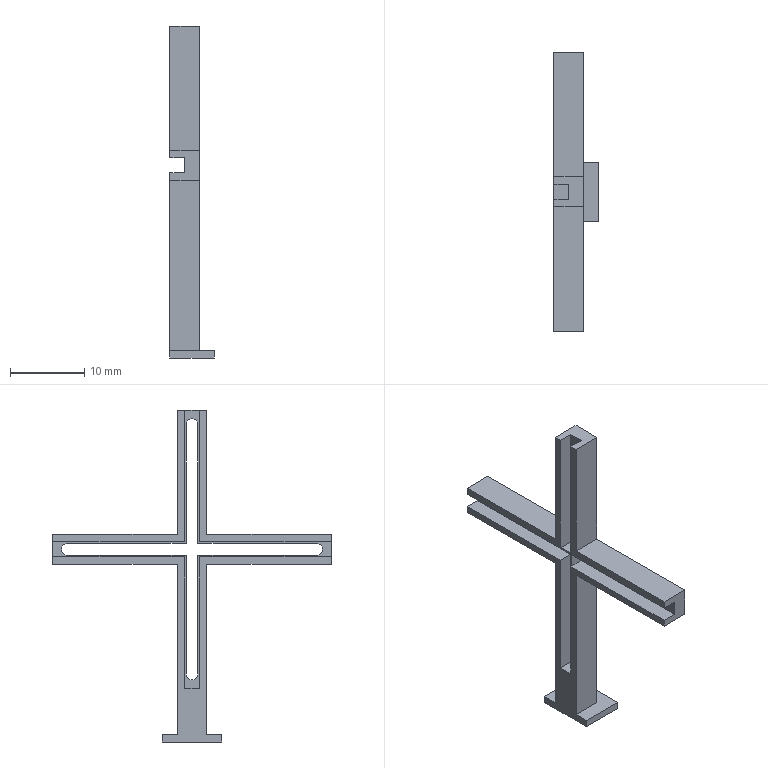Component | NX | CROSS | 1 solid | 42 faces | volume 774 mm3 | plane 38 | cylinder 4 | commonest cylinder face diameters 1.6 x4